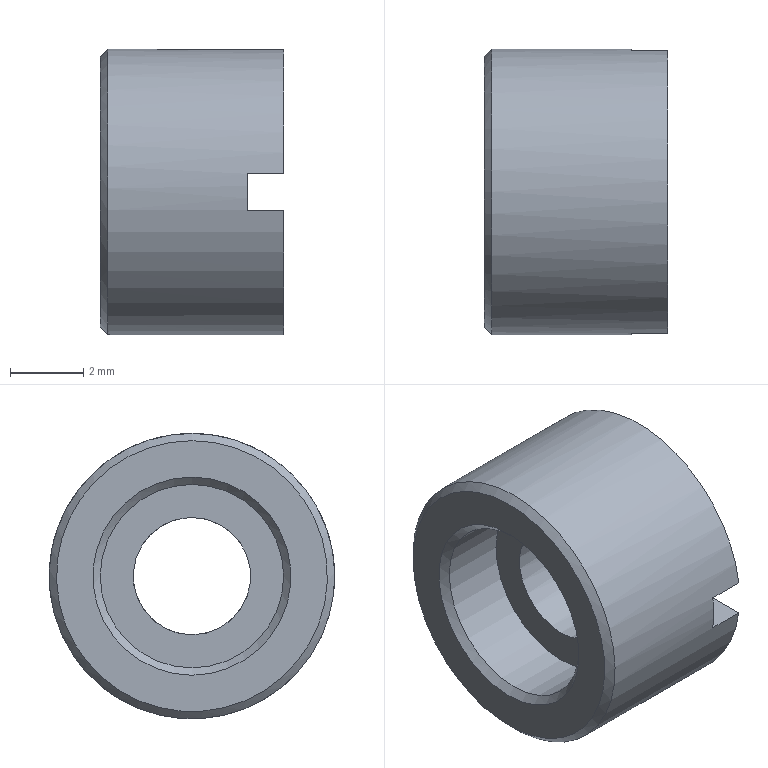Component | NX | HOLED_PLUG | 1 solid | 15 faces | volume 169 mm3 | plane 10 | cylinder 3 | cone 2 | commonest cylinder face diameters 7.785 x1 3.2 x1 5 x1